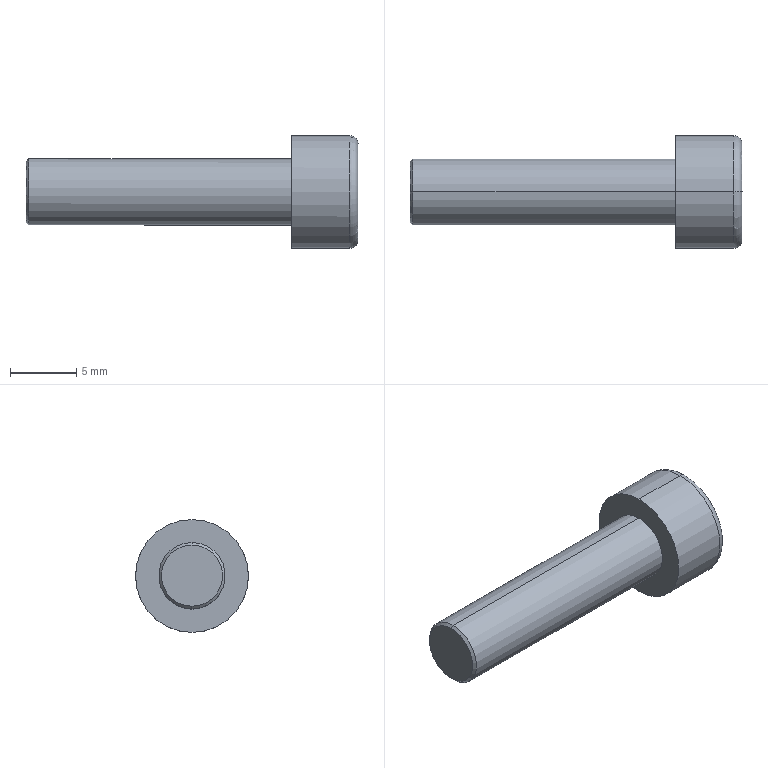Component | SolidWorks | hexagon socket head cap screws gb-94 | 1 solid | 25 faces | box 25.01 x 8.5 x 8.5 mm | volume 634 mm3 | plane 15 | cone 4 | cylinder 4 | torus 2 | commonest cylinder face diameters 5 x2 8.5 x2
STEP:
#1=COLOUR_RGB('',0.7922,0.8196,0.9333);
#2=FILL_AREA_STYLE_COLOUR('',#1);
#3=FILL_AREA_STYLE('',(#2));
#4=SURFACE_STYLE_FILL_AREA(#3);
#5=SURFACE_SIDE_STYLE('',(#4));
#6=SURFACE_STYLE_USAGE(.BOTH.,#5);
#7=PRESENTATION_STYLE_ASSIGNMENT((#6));
#8=CARTESIAN_POINT('',(-4.182,36.006,44.056));
#9=VERTEX_POINT('',#8);
#10=CARTESIAN_POINT('',(-4.183,36.006,43.875));
#11=VERTEX_POINT('',#10);
#12=CARTESIAN_POINT('',(-4.182,36.006,43.966));
#13=DIRECTION('',(-1.,-0.,0.00108));
#14=DIRECTION('',(0.00108,-0.,1.));
#15=AXIS2_PLACEMENT_3D('',#12,#13,#14);
#16=CIRCLE('',#15,0.09055);
#17=EDGE_CURVE('',#9,#11,#16,.T.);
#18=ORIENTED_EDGE('',*,*,#17,.F.);
#19=CARTESIAN_POINT('',(-4.174,36.006,44.064));
#20=VERTEX_POINT('',#19);
#21=CARTESIAN_POINT('',(-4.182,36.006,44.056));
#22=DIRECTION('',(0.7079,-0.,0.7063));
#23=VECTOR('',#22,39.37);
#24=LINE('',#21,#23);
#25=EDGE_CURVE('',#9,#20,#24,.T.);
#26=ORIENTED_EDGE('',*,*,#25,.T.);
#27=CARTESIAN_POINT('',(-4.175,36.006,43.867));
#28=VERTEX_POINT('',#27);
#29=CARTESIAN_POINT('',(-4.175,36.006,43.966));
#30=DIRECTION('',(1.,0.,-0.00108));
#31=DIRECTION('',(0.00108,-0.,1.));
#32=AXIS2_PLACEMENT_3D('',#29,#30,#31);
#33=CIRCLE('',#32,0.09843);
#34=EDGE_CURVE('',#28,#20,#33,.T.);
#35=ORIENTED_EDGE('',*,*,#34,.F.);
#36=CARTESIAN_POINT('',(-4.183,36.006,43.875));
#37=DIRECTION('',(0.7063,0.,-0.7079));
#38=VECTOR('',#37,39.37);
#39=LINE('',#36,#38);
#40=EDGE_CURVE('',#11,#28,#39,.T.);
#41=ORIENTED_EDGE('',*,*,#40,.F.);
#42=EDGE_LOOP('',(#18,#26,#35,#41));
#43=FACE_OUTER_BOUND('',#42,.T.);
#44=CARTESIAN_POINT('',(-4.182,36.006,43.966));
#45=DIRECTION('',(1.,0.,-0.00108));
#46=DIRECTION('',(-0.00108,0.,-1.));
#47=AXIS2_PLACEMENT_3D('',#44,#45,#46);
#48=CONICAL_SURFACE('',#47,0.09055,0.7854);
#49=ADVANCED_FACE('',(#43),#48,.T.);
#50=CARTESIAN_POINT('',(-3.198,36.006,43.822));
#51=VERTEX_POINT('',#50);
#52=CARTESIAN_POINT('',(-3.198,36.006,44.107));
#53=VERTEX_POINT('',#52);
#54=CARTESIAN_POINT('',(-3.198,36.006,43.965));
#55=DIRECTION('',(1.,0.,-0.00108));
#56=DIRECTION('',(0.00108,-0.,1.));
#57=AXIS2_PLACEMENT_3D('',#54,#55,#56);
#58=CIRCLE('',#57,0.1427);
#59=EDGE_CURVE('',#51,#53,#58,.T.);
#60=ORIENTED_EDGE('',*,*,#59,.F.);
#61=CARTESIAN_POINT('',(-3.223,36.006,43.797));
#62=VERTEX_POINT('',#61);
#63=CARTESIAN_POINT('',(-3.223,36.006,43.822));
#64=DIRECTION('',(0.,1.,0.));
#65=DIRECTION('',(0.,-0.,1.));
#66=AXIS2_PLACEMENT_3D('',#63,#64,#65);
#67=CIRCLE('',#66,0.02461);
#68=EDGE_CURVE('',#51,#62,#67,.T.);
#69=ORIENTED_EDGE('',*,*,#68,.T.);
#70=CARTESIAN_POINT('',(-3.223,36.006,44.132));
#71=VERTEX_POINT('',#70);
#72=CARTESIAN_POINT('',(-3.223,36.006,43.965));
#73=DIRECTION('',(-1.,-0.,0.00108));
#74=DIRECTION('',(0.00108,-0.,1.));
#75=AXIS2_PLACEMENT_3D('',#72,#73,#74);
#76=CIRCLE('',#75,0.1673);
#77=EDGE_CURVE('',#71,#62,#76,.T.);
#78=ORIENTED_EDGE('',*,*,#77,.F.);
#79=CARTESIAN_POINT('',(-3.223,36.006,44.108));
#80=DIRECTION('',(-0.,-1.,-0.));
#81=DIRECTION('',(0.,0.,-1.));
#82=AXIS2_PLACEMENT_3D('',#79,#80,#81);
#83=CIRCLE('',#82,0.02461);
#84=EDGE_CURVE('',#53,#71,#83,.T.);
#85=ORIENTED_EDGE('',*,*,#84,.F.);
#86=EDGE_LOOP('',(#60,#69,#78,#85));
#87=FACE_OUTER_BOUND('',#86,.T.);
#88=CARTESIAN_POINT('',(-3.223,36.006,43.965));
#89=DIRECTION('',(-1.,-0.,0.00108));
#90=DIRECTION('',(0.00108,-0.,1.));
#91=AXIS2_PLACEMENT_3D('',#88,#89,#90);
#92=TOROIDAL_SURFACE('',#91,0.1427,0.02461);
#93=ADVANCED_FACE('',(#87),#92,.T.);
#94=CARTESIAN_POINT('',(-3.342,36.006,43.965));
#95=VERTEX_POINT('',#94);
#96=CARTESIAN_POINT('',(-3.297,36.006,43.886));
#97=VERTEX_POINT('',#96);
#98=CARTESIAN_POINT('',(-3.297,36.006,43.886));
#99=DIRECTION('',(0.4991,0.,-0.8666));
#100=VECTOR('',#99,39.37);
#101=LINE('',#98,#100);
#102=EDGE_CURVE('',#95,#97,#101,.T.);
#103=ORIENTED_EDGE('',*,*,#102,.F.);
#104=CARTESIAN_POINT('',(-3.297,36.006,44.044));
#105=VERTEX_POINT('',#104);
#106=CARTESIAN_POINT('',(-3.297,36.006,44.044));
#107=DIRECTION('',(0.5009,-0.,0.8655));
#108=VECTOR('',#107,39.37);
#109=LINE('',#106,#108);
#110=EDGE_CURVE('',#95,#105,#109,.T.);
#111=ORIENTED_EDGE('',*,*,#110,.T.);
#112=CARTESIAN_POINT('',(-3.297,35.966,44.033));
#113=VERTEX_POINT('',#112);
#114=CARTESIAN_POINT('',(-3.297,36.006,43.965));
#115=DIRECTION('',(1.,0.,-0.00108));
#116=DIRECTION('',(0.00108,-0.,1.));
#117=AXIS2_PLACEMENT_3D('',#114,#115,#116);
#118=CIRCLE('',#117,0.07874);
#119=EDGE_CURVE('',#105,#113,#118,.T.);
#120=ORIENTED_EDGE('',*,*,#119,.T.);
#121=CARTESIAN_POINT('',(-3.297,35.927,43.965));
#122=VERTEX_POINT('',#121);
#123=CARTESIAN_POINT('',(-3.297,36.006,43.965));
#124=DIRECTION('',(1.,0.,-0.00108));
#125=DIRECTION('',(0.00108,-0.,1.));
#126=AXIS2_PLACEMENT_3D('',#123,#124,#125);
#127=CIRCLE('',#126,0.07874);
#128=EDGE_CURVE('',#113,#122,#127,.T.);
#129=ORIENTED_EDGE('',*,*,#128,.T.);
#130=CARTESIAN_POINT('',(-3.297,35.966,43.897));
#131=VERTEX_POINT('',#130);
#132=CARTESIAN_POINT('',(-3.297,36.006,43.965));
#133=DIRECTION('',(1.,0.,-0.00108));
#134=DIRECTION('',(0.00108,-0.,1.));
#135=AXIS2_PLACEMENT_3D('',#132,#133,#134);
#136=CIRCLE('',#135,0.07874);
#137=EDGE_CURVE('',#122,#131,#136,.T.);
#138=ORIENTED_EDGE('',*,*,#137,.T.);
#139=CARTESIAN_POINT('',(-3.297,36.006,43.965));
#140=DIRECTION('',(1.,0.,-0.00108));
#141=DIRECTION('',(0.00108,-0.,1.));
#142=AXIS2_PLACEMENT_3D('',#139,#140,#141);
#143=CIRCLE('',#142,0.07874);
#144=EDGE_CURVE('',#131,#97,#143,.T.);
#145=ORIENTED_EDGE('',*,*,#144,.T.);
#146=EDGE_LOOP('',(#103,#111,#120,#129,#138,#145));
#147=FACE_OUTER_BOUND('',#146,.T.);
#148=CARTESIAN_POINT('',(-3.297,36.006,43.965));
#149=DIRECTION('',(1.,0.,-0.00108));
#150=DIRECTION('',(-0.00108,0.,-1.));
#151=AXIS2_PLACEMENT_3D('',#148,#149,#150);
#152=CONICAL_SURFACE('',#151,0.07874,1.047);
#153=ADVANCED_FACE('',(#147),#152,.F.);
#154=ORIENTED_EDGE('',*,*,#34,.T.);
#155=CARTESIAN_POINT('',(-3.395,36.006,44.063));
#156=VERTEX_POINT('',#155);
#157=CARTESIAN_POINT('',(-4.182,36.006,44.064));
#158=DIRECTION('',(1.,0.,-0.00108));
#159=VECTOR('',#158,39.37);
#160=LINE('',#157,#159);
#161=EDGE_CURVE('',#20,#156,#160,.T.);
#162=ORIENTED_EDGE('',*,*,#161,.T.);
#163=CARTESIAN_POINT('',(-3.395,36.006,43.867));
#164=VERTEX_POINT('',#163);
#165=CARTESIAN_POINT('',(-3.395,36.006,43.965));
#166=DIRECTION('',(-1.,-0.,0.00108));
#167=DIRECTION('',(0.00108,-0.,1.));
#168=AXIS2_PLACEMENT_3D('',#165,#166,#167);
#169=CIRCLE('',#168,0.09843);
#170=EDGE_CURVE('',#156,#164,#169,.T.);
#171=ORIENTED_EDGE('',*,*,#170,.T.);
#172=CARTESIAN_POINT('',(-4.183,36.006,43.867));
#173=DIRECTION('',(1.,0.,-0.00108));
#174=VECTOR('',#173,39.37);
#175=LINE('',#172,#174);
#176=EDGE_CURVE('',#28,#164,#175,.T.);
#177=ORIENTED_EDGE('',*,*,#176,.F.);
#178=EDGE_LOOP('',(#154,#162,#171,#177));
#179=FACE_OUTER_BOUND('',#178,.T.);
#180=CARTESIAN_POINT('',(-4.182,36.006,43.966));
#181=DIRECTION('',(1.,0.,-0.00108));
#182=DIRECTION('',(-0.00108,0.,-1.));
#183=AXIS2_PLACEMENT_3D('',#180,#181,#182);
#184=CYLINDRICAL_SURFACE('',#183,0.09843);
#185=ADVANCED_FACE('',(#179),#184,.T.);
#186=CARTESIAN_POINT('',(-3.395,36.006,44.132));
#187=VERTEX_POINT('',#186);
#188=CARTESIAN_POINT('',(-3.395,36.006,43.798));
#189=VERTEX_POINT('',#188);
#190=CARTESIAN_POINT('',(-3.395,36.006,43.965));
#191=DIRECTION('',(-1.,-0.,0.00108));
#192=DIRECTION('',(0.00108,-0.,1.));
#193=AXIS2_PLACEMENT_3D('',#190,#191,#192);
#194=CIRCLE('',#193,0.1673);
#195=EDGE_CURVE('',#187,#189,#194,.T.);
#196=ORIENTED_EDGE('',*,*,#195,.F.);
#197=CARTESIAN_POINT('',(-3.395,36.006,44.132));
#198=DIRECTION('',(1.,0.,-0.00108));
#199=VECTOR('',#198,39.37);
#200=LINE('',#197,#199);
#201=EDGE_CURVE('',#187,#71,#200,.T.);
#202=ORIENTED_EDGE('',*,*,#201,.T.);
#203=ORIENTED_EDGE('',*,*,#77,.T.);
#204=CARTESIAN_POINT('',(-3.395,36.006,43.798));
#205=DIRECTION('',(1.,0.,-0.00108));
#206=VECTOR('',#205,39.37);
#207=LINE('',#204,#206);
#208=EDGE_CURVE('',#189,#62,#207,.T.);
#209=ORIENTED_EDGE('',*,*,#208,.F.);
#210=EDGE_LOOP('',(#196,#202,#203,#209));
#211=FACE_OUTER_BOUND('',#210,.T.);
#212=CARTESIAN_POINT('',(-3.395,36.006,43.965));
#213=DIRECTION('',(1.,0.,-0.00108));
#214=DIRECTION('',(-0.00108,0.,-1.));
#215=AXIS2_PLACEMENT_3D('',#212,#213,#214);
#216=CYLINDRICAL_SURFACE('',#215,0.1673);
#217=ADVANCED_FACE('',(#211),#216,.T.);
#218=ORIENTED_EDGE('',*,*,#128,.F.);
#219=CARTESIAN_POINT('',(-3.297,35.927,44.01));
#220=VERTEX_POINT('',#219);
#221=CARTESIAN_POINT('',(-3.297,35.927,44.01));
#222=DIRECTION('',(0.0005402,0.866,0.5));
#223=VECTOR('',#222,39.37);
#224=LINE('',#221,#223);
#225=EDGE_CURVE('',#220,#113,#224,.T.);
#226=ORIENTED_EDGE('',*,*,#225,.F.);
#227=CARTESIAN_POINT('',(-3.297,35.927,43.919));
#228=DIRECTION('',(0.00108,-0.,1.));
#229=VECTOR('',#228,39.37);
#230=LINE('',#227,#229);
#231=EDGE_CURVE('',#122,#220,#230,.T.);
#232=ORIENTED_EDGE('',*,*,#231,.F.);
#233=EDGE_LOOP('',(#218,#226,#232));
#234=FACE_OUTER_BOUND('',#233,.T.);
#235=CARTESIAN_POINT('',(-3.296,36.084,44.101));
#236=DIRECTION('',(-1.,-0.,0.00108));
#237=DIRECTION('',(0.00108,-0.,1.));
#238=AXIS2_PLACEMENT_3D('',#235,#236,#237);
#239=PLANE('',#238);
#240=ADVANCED_FACE('',(#234),#239,.F.);
#241=ORIENTED_EDGE('',*,*,#137,.F.);
#242=CARTESIAN_POINT('',(-3.297,35.927,43.919));
#243=VERTEX_POINT('',#242);
#244=CARTESIAN_POINT('',(-3.297,35.927,43.919));
#245=DIRECTION('',(0.00108,-0.,1.));
#246=VECTOR('',#245,39.37);
#247=LINE('',#244,#246);
#248=EDGE_CURVE('',#243,#122,#247,.T.);
#249=ORIENTED_EDGE('',*,*,#248,.F.);
#250=CARTESIAN_POINT('',(-3.297,36.006,43.874));
#251=DIRECTION('',(0.0005402,-0.866,0.5));
#252=VECTOR('',#251,39.37);
#253=LINE('',#250,#252);
#254=EDGE_CURVE('',#131,#243,#253,.T.);
#255=ORIENTED_EDGE('',*,*,#254,.F.);
#256=EDGE_LOOP('',(#241,#249,#255));
#257=FACE_OUTER_BOUND('',#256,.T.);
#258=CARTESIAN_POINT('',(-3.296,36.084,44.101));
#259=DIRECTION('',(-1.,-0.,0.00108));
#260=DIRECTION('',(0.00108,-0.,1.));
#261=AXIS2_PLACEMENT_3D('',#258,#259,#260);
#262=PLANE('',#261);
#263=ADVANCED_FACE('',(#257),#262,.F.);
#264=ORIENTED_EDGE('',*,*,#144,.F.);
#265=CARTESIAN_POINT('',(-3.297,36.006,43.874));
#266=VERTEX_POINT('',#265);
#267=CARTESIAN_POINT('',(-3.297,36.006,43.874));
#268=DIRECTION('',(0.0005402,-0.866,0.5));
#269=VECTOR('',#268,39.37);
#270=LINE('',#267,#269);
#271=EDGE_CURVE('',#266,#131,#270,.T.);
#272=ORIENTED_EDGE('',*,*,#271,.F.);
#273=CARTESIAN_POINT('',(-3.297,36.045,43.897));
#274=VERTEX_POINT('',#273);
#275=CARTESIAN_POINT('',(-3.297,36.084,43.919));
#276=DIRECTION('',(-0.0005402,-0.866,-0.5));
#277=VECTOR('',#276,39.37);
#278=LINE('',#275,#277);
#279=EDGE_CURVE('',#274,#266,#278,.T.);
#280=ORIENTED_EDGE('',*,*,#279,.F.);
#281=CARTESIAN_POINT('',(-3.297,36.006,43.965));
#282=DIRECTION('',(1.,0.,-0.00108));
#283=DIRECTION('',(0.00108,-0.,1.));
#284=AXIS2_PLACEMENT_3D('',#281,#282,#283);
#285=CIRCLE('',#284,0.07874);
#286=EDGE_CURVE('',#97,#274,#285,.T.);
#287=ORIENTED_EDGE('',*,*,#286,.F.);
#288=EDGE_LOOP('',(#264,#272,#280,#287));
#289=FACE_OUTER_BOUND('',#288,.T.);
#290=CARTESIAN_POINT('',(-3.296,36.084,44.101));
#291=DIRECTION('',(-1.,-0.,0.00108));
#292=DIRECTION('',(0.00108,-0.,1.));
#293=AXIS2_PLACEMENT_3D('',#290,#291,#292);
#294=PLANE('',#293);
#295=ADVANCED_FACE('',(#289),#294,.F.);
#296=CARTESIAN_POINT('',(-3.297,36.084,43.965));
#297=VERTEX_POINT('',#296);
#298=CARTESIAN_POINT('',(-3.297,36.006,43.965));
#299=DIRECTION('',(1.,0.,-0.00108));
#300=DIRECTION('',(0.00108,-0.,1.));
#301=AXIS2_PLACEMENT_3D('',#298,#299,#300);
#302=CIRCLE('',#301,0.07874);
#303=EDGE_CURVE('',#274,#297,#302,.T.);
#304=ORIENTED_EDGE('',*,*,#303,.F.);
#305=CARTESIAN_POINT('',(-3.297,36.084,43.919));
#306=VERTEX_POINT('',#305);
#307=CARTESIAN_POINT('',(-3.297,36.084,43.919));
#308=DIRECTION('',(-0.0005402,-0.866,-0.5));
#309=VECTOR('',#308,39.37);
#310=LINE('',#307,#309);
#311=EDGE_CURVE('',#306,#274,#310,.T.);
#312=ORIENTED_EDGE('',*,*,#311,.F.);
#313=CARTESIAN_POINT('',(-3.297,36.084,44.01));
#314=DIRECTION('',(-0.00108,0.,-1.));
#315=VECTOR('',#314,39.37);
#316=LINE('',#313,#315);
#317=EDGE_CURVE('',#297,#306,#316,.T.);
#318=ORIENTED_EDGE('',*,*,#317,.F.);
#319=EDGE_LOOP('',(#304,#312,#318));
#320=FACE_OUTER_BOUND('',#319,.T.);
#321=CARTESIAN_POINT('',(-3.296,36.084,44.101));
#322=DIRECTION('',(-1.,-0.,0.00108));
#323=DIRECTION('',(0.00108,-0.,1.));
#324=AXIS2_PLACEMENT_3D('',#321,#322,#323);
#325=PLANE('',#324);
#326=ADVANCED_FACE('',(#320),#325,.F.);
#327=CARTESIAN_POINT('',(-3.297,36.045,44.033));
#328=VERTEX_POINT('',#327);
#329=CARTESIAN_POINT('',(-3.297,36.006,43.965));
#330=DIRECTION('',(-1.,-0.,0.00108));
#331=DIRECTION('',(0.00108,-0.,1.));
#332=AXIS2_PLACEMENT_3D('',#329,#330,#331);
#333=CIRCLE('',#332,0.07874);
#334=EDGE_CURVE('',#328,#297,#333,.T.);
#335=ORIENTED_EDGE('',*,*,#334,.T.);
#336=CARTESIAN_POINT('',(-3.297,36.084,44.01));
#337=VERTEX_POINT('',#336);
#338=CARTESIAN_POINT('',(-3.297,36.084,44.01));
#339=DIRECTION('',(-0.00108,0.,-1.));
#340=VECTOR('',#339,39.37);
#341=LINE('',#338,#340);
#342=EDGE_CURVE('',#337,#297,#341,.T.);
#343=ORIENTED_EDGE('',*,*,#342,.F.);
#344=CARTESIAN_POINT('',(-3.297,36.006,44.056));
#345=DIRECTION('',(-0.0005402,0.866,-0.5));
#346=VECTOR('',#345,39.37);
#347=LINE('',#344,#346);
#348=EDGE_CURVE('',#328,#337,#347,.T.);
#349=ORIENTED_EDGE('',*,*,#348,.F.);
#350=EDGE_LOOP('',(#335,#343,#349));
#351=FACE_OUTER_BOUND('',#350,.T.);
#352=CARTESIAN_POINT('',(-3.296,36.084,44.101));
#353=DIRECTION('',(-1.,-0.,0.00108));
#354=DIRECTION('',(0.00108,-0.,1.));
#355=AXIS2_PLACEMENT_3D('',#352,#353,#354);
#356=PLANE('',#355);
#357=ADVANCED_FACE('',(#351),#356,.F.);
#358=CARTESIAN_POINT('',(-3.297,36.006,43.965));
#359=DIRECTION('',(1.,0.,-0.00108));
#360=DIRECTION('',(0.00108,-0.,1.));
#361=AXIS2_PLACEMENT_3D('',#358,#359,#360);
#362=CIRCLE('',#361,0.07874);
#363=EDGE_CURVE('',#328,#105,#362,.T.);
#364=ORIENTED_EDGE('',*,*,#363,.F.);
#365=CARTESIAN_POINT('',(-3.297,36.006,44.056));
#366=VERTEX_POINT('',#365);
#367=CARTESIAN_POINT('',(-3.297,36.006,44.056));
#368=DIRECTION('',(-0.0005402,0.866,-0.5));
#369=VECTOR('',#368,39.37);
#370=LINE('',#367,#369);
#371=EDGE_CURVE('',#366,#328,#370,.T.);
#372=ORIENTED_EDGE('',*,*,#371,.F.);
#373=CARTESIAN_POINT('',(-3.297,35.927,44.01));
#374=DIRECTION('',(0.0005402,0.866,0.5));
#375=VECTOR('',#374,39.37);
#376=LINE('',#373,#375);
#377=EDGE_CURVE('',#113,#366,#376,.T.);
#378=ORIENTED_EDGE('',*,*,#377,.F.);
#379=ORIENTED_EDGE('',*,*,#119,.F.);
#380=EDGE_LOOP('',(#364,#372,#378,#379));
#381=FACE_OUTER_BOUND('',#380,.T.);
#382=CARTESIAN_POINT('',(-3.296,36.084,44.101));
#383=DIRECTION('',(-1.,-0.,0.00108));
#384=DIRECTION('',(0.00108,-0.,1.));
#385=AXIS2_PLACEMENT_3D('',#382,#383,#384);
#386=PLANE('',#385);
#387=ADVANCED_FACE('',(#381),#386,.F.);
#388=CARTESIAN_POINT('',(-3.198,36.006,43.965));
#389=DIRECTION('',(1.,0.,-0.00108));
#390=DIRECTION('',(0.00108,-0.,1.));
#391=AXIS2_PLACEMENT_3D('',#388,#389,#390);
#392=CIRCLE('',#391,0.1427);
#393=EDGE_CURVE('',#53,#51,#392,.T.);
#394=ORIENTED_EDGE('',*,*,#393,.T.);
#395=ORIENTED_EDGE('',*,*,#59,.T.);
#396=EDGE_LOOP('',(#394,#395));
#397=FACE_OUTER_BOUND('',#396,.T.);
#398=CARTESIAN_POINT('',(-3.198,35.927,44.01));
#399=VERTEX_POINT('',#398);
#400=CARTESIAN_POINT('',(-3.198,36.006,44.056));
#401=VERTEX_POINT('',#400);
#402=CARTESIAN_POINT('',(-3.198,35.927,44.01));
#403=DIRECTION('',(0.0005402,0.866,0.5));
#404=VECTOR('',#403,39.37);
#405=LINE('',#402,#404);
#406=EDGE_CURVE('',#399,#401,#405,.T.);
#407=ORIENTED_EDGE('',*,*,#406,.T.);
#408=CARTESIAN_POINT('',(-3.198,36.084,44.01));
#409=VERTEX_POINT('',#408);
#410=CARTESIAN_POINT('',(-3.198,36.006,44.056));
#411=DIRECTION('',(-0.0005402,0.866,-0.5));
#412=VECTOR('',#411,39.37);
#413=LINE('',#410,#412);
#414=EDGE_CURVE('',#401,#409,#413,.T.);
#415=ORIENTED_EDGE('',*,*,#414,.T.);
#416=CARTESIAN_POINT('',(-3.198,36.084,43.919));
#417=VERTEX_POINT('',#416);
#418=CARTESIAN_POINT('',(-3.198,36.084,44.01));
#419=DIRECTION('',(-0.00108,0.,-1.));
#420=VECTOR('',#419,39.37);
#421=LINE('',#418,#420);
#422=EDGE_CURVE('',#409,#417,#421,.T.);
#423=ORIENTED_EDGE('',*,*,#422,.T.);
#424=CARTESIAN_POINT('',(-3.198,36.006,43.874));
#425=VERTEX_POINT('',#424);
#426=CARTESIAN_POINT('',(-3.198,36.084,43.919));
#427=DIRECTION('',(-0.0005402,-0.866,-0.5));
#428=VECTOR('',#427,39.37);
#429=LINE('',#426,#428);
#430=EDGE_CURVE('',#417,#425,#429,.T.);
#431=ORIENTED_EDGE('',*,*,#430,.T.);
#432=CARTESIAN_POINT('',(-3.198,35.927,43.919));
#433=VERTEX_POINT('',#432);
#434=CARTESIAN_POINT('',(-3.198,36.006,43.874));
#435=DIRECTION('',(0.0005402,-0.866,0.5));
#436=VECTOR('',#435,39.37);
#437=LINE('',#434,#436);
#438=EDGE_CURVE('',#425,#433,#437,.T.);
#439=ORIENTED_EDGE('',*,*,#438,.T.);
#440=CARTESIAN_POINT('',(-3.198,35.927,43.919));
#441=DIRECTION('',(0.00108,-0.,1.));
#442=VECTOR('',#441,39.37);
#443=LINE('',#440,#442);
#444=EDGE_CURVE('',#433,#399,#443,.T.);
#445=ORIENTED_EDGE('',*,*,#444,.T.);
#446=EDGE_LOOP('',(#407,#415,#423,#431,#439,#445));
#447=FACE_BOUND('',#446,.T.);
#448=CARTESIAN_POINT('',(-3.198,36.006,43.965));
#449=DIRECTION('',(-1.,-0.,0.00108));
#450=DIRECTION('',(0.00108,-0.,1.));
#451=AXIS2_PLACEMENT_3D('',#448,#449,#450);
#452=PLANE('',#451);
#453=ADVANCED_FACE('',(#397,#447),#452,.F.);
#454=CARTESIAN_POINT('',(-3.395,36.006,43.965));
#455=DIRECTION('',(-1.,-0.,0.00108));
#456=DIRECTION('',(0.00108,-0.,1.));
#457=AXIS2_PLACEMENT_3D('',#454,#455,#456);
#458=CIRCLE('',#457,0.1673);
#459=EDGE_CURVE('',#189,#187,#458,.T.);
#460=ORIENTED_EDGE('',*,*,#459,.T.);
#461=ORIENTED_EDGE('',*,*,#195,.T.);
#462=EDGE_LOOP('',(#460,#461));
#463=FACE_OUTER_BOUND('',#462,.T.);
#464=CARTESIAN_POINT('',(-3.395,36.006,43.965));
#465=DIRECTION('',(-1.,-0.,0.00108));
#466=DIRECTION('',(0.00108,-0.,1.));
#467=AXIS2_PLACEMENT_3D('',#464,#465,#466);
#468=CIRCLE('',#467,0.09843);
#469=EDGE_CURVE('',#164,#156,#468,.T.);
#470=ORIENTED_EDGE('',*,*,#469,.F.);
#471=ORIENTED_EDGE('',*,*,#170,.F.);
#472=EDGE_LOOP('',(#470,#471));
#473=FACE_BOUND('',#472,.T.);
#474=CARTESIAN_POINT('',(-3.395,36.006,43.965));
#475=DIRECTION('',(-1.,-0.,0.00108));
#476=DIRECTION('',(0.00108,-0.,1.));
#477=AXIS2_PLACEMENT_3D('',#474,#475,#476);
#478=PLANE('',#477);
#479=ADVANCED_FACE('',(#463,#473),#478,.T.);
#480=ORIENTED_EDGE('',*,*,#201,.F.);
#481=ORIENTED_EDGE('',*,*,#459,.F.);
#482=ORIENTED_EDGE('',*,*,#208,.T.);
#483=CARTESIAN_POINT('',(-3.223,36.006,43.965));
#484=DIRECTION('',(-1.,-0.,0.00108));
#485=DIRECTION('',(0.00108,-0.,1.));
#486=AXIS2_PLACEMENT_3D('',#483,#484,#485);
#487=CIRCLE('',#486,0.1673);
#488=EDGE_CURVE('',#62,#71,#487,.T.);
#489=ORIENTED_EDGE('',*,*,#488,.T.);
#490=EDGE_LOOP('',(#480,#481,#482,#489));
#491=FACE_OUTER_BOUND('',#490,.T.);
#492=CARTESIAN_POINT('',(-3.395,36.006,43.965));
#493=DIRECTION('',(1.,0.,-0.00108));
#494=DIRECTION('',(-0.00108,0.,-1.));
#495=AXIS2_PLACEMENT_3D('',#492,#493,#494);
#496=CYLINDRICAL_SURFACE('',#495,0.1673);
#497=ADVANCED_FACE('',(#491),#496,.T.);
#498=ORIENTED_EDGE('',*,*,#161,.F.);
#499=CARTESIAN_POINT('',(-4.175,36.006,43.966));
#500=DIRECTION('',(1.,0.,-0.00108));
#501=DIRECTION('',(0.00108,-0.,1.));
#502=AXIS2_PLACEMENT_3D('',#499,#500,#501);
#503=CIRCLE('',#502,0.09843);
#504=EDGE_CURVE('',#20,#28,#503,.T.);
#505=ORIENTED_EDGE('',*,*,#504,.T.);
#506=ORIENTED_EDGE('',*,*,#176,.T.);
#507=ORIENTED_EDGE('',*,*,#469,.T.);
#508=EDGE_LOOP('',(#498,#505,#506,#507));
#509=FACE_OUTER_BOUND('',#508,.T.);
#510=CARTESIAN_POINT('',(-4.182,36.006,43.966));
#511=DIRECTION('',(1.,0.,-0.00108));
#512=DIRECTION('',(-0.00108,0.,-1.));
#513=AXIS2_PLACEMENT_3D('',#510,#511,#512);
#514=CYLINDRICAL_SURFACE('',#513,0.09843);
#515=ADVANCED_FACE('',(#509),#514,.T.);
#516=CARTESIAN_POINT('',(-4.182,36.006,43.966));
#517=DIRECTION('',(-1.,-0.,0.00108));
#518=DIRECTION('',(0.00108,-0.,1.));
#519=AXIS2_PLACEMENT_3D('',#516,#517,#518);
#520=CIRCLE('',#519,0.09055);
#521=EDGE_CURVE('',#11,#9,#520,.T.);
#522=ORIENTED_EDGE('',*,*,#521,.T.);
#523=ORIENTED_EDGE('',*,*,#17,.T.);
#524=EDGE_LOOP('',(#522,#523));
#525=FACE_OUTER_BOUND('',#524,.T.);
#526=CARTESIAN_POINT('',(-4.182,36.006,43.966));
#527=DIRECTION('',(-1.,-0.,0.00108));
#528=DIRECTION('',(0.00108,-0.,1.));
#529=AXIS2_PLACEMENT_3D('',#526,#527,#528);
#530=PLANE('',#529);
#531=ADVANCED_FACE('',(#525),#530,.T.);
#532=ORIENTED_EDGE('',*,*,#406,.F.);
#533=CARTESIAN_POINT('',(-3.297,35.927,44.01));
#534=DIRECTION('',(1.,0.,-0.00108));
#535=VECTOR('',#534,39.37);
#536=LINE('',#533,#535);
#537=EDGE_CURVE('',#220,#399,#536,.T.);
#538=ORIENTED_EDGE('',*,*,#537,.F.);
#539=ORIENTED_EDGE('',*,*,#225,.T.);
#540=ORIENTED_EDGE('',*,*,#377,.T.);
#541=CARTESIAN_POINT('',(-3.297,36.006,44.056));
#542=DIRECTION('',(1.,0.,-0.00108));
#543=VECTOR('',#542,39.37);
#544=LINE('',#541,#543);
#545=EDGE_CURVE('',#366,#401,#544,.T.);
#546=ORIENTED_EDGE('',*,*,#545,.T.);
#547=EDGE_LOOP('',(#532,#538,#539,#540,#546));
#548=FACE_OUTER_BOUND('',#547,.T.);
#549=CARTESIAN_POINT('',(-3.297,35.927,44.01));
#550=DIRECTION('',(-0.0009357,0.5,-0.866));
#551=DIRECTION('',(-0.0005402,-0.866,-0.5));
#552=AXIS2_PLACEMENT_3D('',#549,#550,#551);
#553=PLANE('',#552);
#554=ADVANCED_FACE('',(#548),#553,.T.);
#555=ORIENTED_EDGE('',*,*,#414,.F.);
#556=ORIENTED_EDGE('',*,*,#545,.F.);
#557=ORIENTED_EDGE('',*,*,#371,.T.);
#558=ORIENTED_EDGE('',*,*,#348,.T.);
#559=CARTESIAN_POINT('',(-3.297,36.084,44.01));
#560=DIRECTION('',(1.,0.,-0.00108));
#561=VECTOR('',#560,39.37);
#562=LINE('',#559,#561);
#563=EDGE_CURVE('',#337,#409,#562,.T.);
#564=ORIENTED_EDGE('',*,*,#563,.T.);
#565=EDGE_LOOP('',(#555,#556,#557,#558,#564));
#566=FACE_OUTER_BOUND('',#565,.T.);
#567=CARTESIAN_POINT('',(-3.297,36.006,44.056));
#568=DIRECTION('',(-0.0009357,-0.5,-0.866));
#569=DIRECTION('',(0.0005402,-0.866,0.5));
#570=AXIS2_PLACEMENT_3D('',#567,#568,#569);
#571=PLANE('',#570);
#572=ADVANCED_FACE('',(#566),#571,.T.);
#573=ORIENTED_EDGE('',*,*,#422,.F.);
#574=ORIENTED_EDGE('',*,*,#563,.F.);
#575=ORIENTED_EDGE('',*,*,#342,.T.);
#576=ORIENTED_EDGE('',*,*,#317,.T.);
#577=CARTESIAN_POINT('',(-3.297,36.084,43.919));
#578=DIRECTION('',(1.,0.,-0.00108));
#579=VECTOR('',#578,39.37);
#580=LINE('',#577,#579);
#581=EDGE_CURVE('',#306,#417,#580,.T.);
#582=ORIENTED_EDGE('',*,*,#581,.T.);
#583=EDGE_LOOP('',(#573,#574,#575,#576,#582));
#584=FACE_OUTER_BOUND('',#583,.T.);
#585=CARTESIAN_POINT('',(-3.297,36.084,44.01));
#586=DIRECTION('',(-0.,-1.,-0.));
#587=DIRECTION('',(0.00108,-0.,1.));
#588=AXIS2_PLACEMENT_3D('',#585,#586,#587);
#589=PLANE('',#588);
#590=ADVANCED_FACE('',(#584),#589,.T.);
#591=ORIENTED_EDGE('',*,*,#430,.F.);
#592=ORIENTED_EDGE('',*,*,#581,.F.);
#593=ORIENTED_EDGE('',*,*,#311,.T.);
#594=ORIENTED_EDGE('',*,*,#279,.T.);
#595=CARTESIAN_POINT('',(-3.297,36.006,43.874));
#596=DIRECTION('',(1.,0.,-0.00108));
#597=VECTOR('',#596,39.37);
#598=LINE('',#595,#597);
#599=EDGE_CURVE('',#266,#425,#598,.T.);
#600=ORIENTED_EDGE('',*,*,#599,.T.);
#601=EDGE_LOOP('',(#591,#592,#593,#594,#600));
#602=FACE_OUTER_BOUND('',#601,.T.);
#603=CARTESIAN_POINT('',(-3.297,36.084,43.919));
#604=DIRECTION('',(0.0009357,-0.5,0.866));
#605=DIRECTION('',(0.0005402,0.866,0.5));
#606=AXIS2_PLACEMENT_3D('',#603,#604,#605);
#607=PLANE('',#606);
#608=ADVANCED_FACE('',(#602),#607,.T.);
#609=ORIENTED_EDGE('',*,*,#438,.F.);
#610=ORIENTED_EDGE('',*,*,#599,.F.);
#611=ORIENTED_EDGE('',*,*,#271,.T.);
#612=ORIENTED_EDGE('',*,*,#254,.T.);
#613=CARTESIAN_POINT('',(-3.297,35.927,43.919));
#614=DIRECTION('',(1.,0.,-0.00108));
#615=VECTOR('',#614,39.37);
#616=LINE('',#613,#615);
#617=EDGE_CURVE('',#243,#433,#616,.T.);
#618=ORIENTED_EDGE('',*,*,#617,.T.);
#619=EDGE_LOOP('',(#609,#610,#611,#612,#618));
#620=FACE_OUTER_BOUND('',#619,.T.);
#621=CARTESIAN_POINT('',(-3.297,36.006,43.874));
#622=DIRECTION('',(0.0009357,0.5,0.866));
#623=DIRECTION('',(-0.0005402,0.866,-0.5));
#624=AXIS2_PLACEMENT_3D('',#621,#622,#623);
#625=PLANE('',#624);
#626=ADVANCED_FACE('',(#620),#625,.T.);
#627=ORIENTED_EDGE('',*,*,#444,.F.);
#628=ORIENTED_EDGE('',*,*,#617,.F.);
#629=ORIENTED_EDGE('',*,*,#248,.T.);
#630=ORIENTED_EDGE('',*,*,#231,.T.);
#631=ORIENTED_EDGE('',*,*,#537,.T.);
#632=EDGE_LOOP('',(#627,#628,#629,#630,#631));
#633=FACE_OUTER_BOUND('',#632,.T.);
#634=CARTESIAN_POINT('',(-3.297,35.927,43.919));
#635=DIRECTION('',(0.,1.,0.));
#636=DIRECTION('',(-0.00108,0.,-1.));
#637=AXIS2_PLACEMENT_3D('',#634,#635,#636);
#638=PLANE('',#637);
#639=ADVANCED_FACE('',(#633),#638,.T.);
#640=ORIENTED_EDGE('',*,*,#110,.F.);
#641=ORIENTED_EDGE('',*,*,#102,.T.);
#642=ORIENTED_EDGE('',*,*,#286,.T.);
#643=ORIENTED_EDGE('',*,*,#303,.T.);
#644=ORIENTED_EDGE('',*,*,#334,.F.);
#645=ORIENTED_EDGE('',*,*,#363,.T.);
#646=EDGE_LOOP('',(#640,#641,#642,#643,#644,#645));
#647=FACE_OUTER_BOUND('',#646,.T.);
#648=CARTESIAN_POINT('',(-3.297,36.006,43.965));
#649=DIRECTION('',(1.,0.,-0.00108));
#650=DIRECTION('',(-0.00108,0.,-1.));
#651=AXIS2_PLACEMENT_3D('',#648,#649,#650);
#652=CONICAL_SURFACE('',#651,0.07874,1.047);
#653=ADVANCED_FACE('',(#647),#652,.F.);
#654=ORIENTED_EDGE('',*,*,#68,.F.);
#655=ORIENTED_EDGE('',*,*,#393,.F.);
#656=ORIENTED_EDGE('',*,*,#84,.T.);
#657=ORIENTED_EDGE('',*,*,#488,.F.);
#658=EDGE_LOOP('',(#654,#655,#656,#657));
#659=FACE_OUTER_BOUND('',#658,.T.);
#660=CARTESIAN_POINT('',(-3.223,36.006,43.965));
#661=DIRECTION('',(-1.,-0.,0.00108));
#662=DIRECTION('',(0.00108,-0.,1.));
#663=AXIS2_PLACEMENT_3D('',#660,#661,#662);
#664=TOROIDAL_SURFACE('',#663,0.1427,0.02461);
#665=ADVANCED_FACE('',(#659),#664,.T.);
#666=ORIENTED_EDGE('',*,*,#25,.F.);
#667=ORIENTED_EDGE('',*,*,#521,.F.);
#668=ORIENTED_EDGE('',*,*,#40,.T.);
#669=ORIENTED_EDGE('',*,*,#504,.F.);
#670=EDGE_LOOP('',(#666,#667,#668,#669));
#671=FACE_OUTER_BOUND('',#670,.T.);
#672=CARTESIAN_POINT('',(-4.182,36.006,43.966));
#673=DIRECTION('',(1.,0.,-0.00108));
#674=DIRECTION('',(-0.00108,0.,-1.));
#675=AXIS2_PLACEMENT_3D('',#672,#673,#674);
#676=CONICAL_SURFACE('',#675,0.09055,0.7854);
#677=ADVANCED_FACE('',(#671),#676,.T.);
#678=CLOSED_SHELL('',(#49,#93,#153,#185,#217,#240,#263,#295,#326,#357,#387,#453,#479,#497,#515,#531,#554,#572,#590,#608,#626,#639,#653,#665,#677));
#679=MANIFOLD_SOLID_BREP('',#678);
#680=STYLED_ITEM('',(#7),#679);
#681=PRESENTATION_LAYER_ASSIGNMENT('','',(#680));
#682=CARTESIAN_POINT('',(0.,0.,0.));
#683=DIRECTION('',(0.,0.,1.));
#684=DIRECTION('',(1.,0.,0.));
#685=AXIS2_PLACEMENT_3D('',#682,#683,#684);
#686=(LENGTH_UNIT()NAMED_UNIT(*)SI_UNIT($,.METRE.));
#687=LENGTH_MEASURE_WITH_UNIT(LENGTH_MEASURE(0.0254),#686);
#688=DIMENSIONAL_EXPONENTS(1.,0.,0.,0.,0.,0.,0.);
#689=(CONVERSION_BASED_UNIT('',#687)LENGTH_UNIT()NAMED_UNIT(#688));
#690=UNCERTAINTY_MEASURE_WITH_UNIT(LENGTH_MEASURE(0.00001),#689,'','');
#691=(NAMED_UNIT(*)PLANE_ANGLE_UNIT()SI_UNIT($,.RADIAN.));
#692=(NAMED_UNIT(*)SI_UNIT($,.STERADIAN.)SOLID_ANGLE_UNIT());
#693=(GEOMETRIC_REPRESENTATION_CONTEXT(3)GLOBAL_UNCERTAINTY_ASSIGNED_CONTEXT((#690))GLOBAL_UNIT_ASSIGNED_CONTEXT((#689,#691,#692))REPRESENTATION_CONTEXT('',''));
#694=ADVANCED_BREP_SHAPE_REPRESENTATION('',(#679,#685),#693);
#695=(LENGTH_UNIT()NAMED_UNIT(*)SI_UNIT($,.METRE.));
#696=LENGTH_MEASURE_WITH_UNIT(LENGTH_MEASURE(0.0254),#695);
#697=DIMENSIONAL_EXPONENTS(1.,0.,0.,0.,0.,0.,0.);
#698=(CONVERSION_BASED_UNIT('',#696)LENGTH_UNIT()NAMED_UNIT(#697));
#699=UNCERTAINTY_MEASURE_WITH_UNIT(LENGTH_MEASURE(0.00001),#698,'','');
#700=(NAMED_UNIT(*)PLANE_ANGLE_UNIT()SI_UNIT($,.RADIAN.));
#701=(NAMED_UNIT(*)SI_UNIT($,.STERADIAN.)SOLID_ANGLE_UNIT());
#702=(GEOMETRIC_REPRESENTATION_CONTEXT(3)GLOBAL_UNCERTAINTY_ASSIGNED_CONTEXT((#699))GLOBAL_UNIT_ASSIGNED_CONTEXT((#698,#700,#701))REPRESENTATION_CONTEXT('',''));
#703=MECHANICAL_DESIGN_GEOMETRIC_PRESENTATION_REPRESENTATION('',(#680),#702);